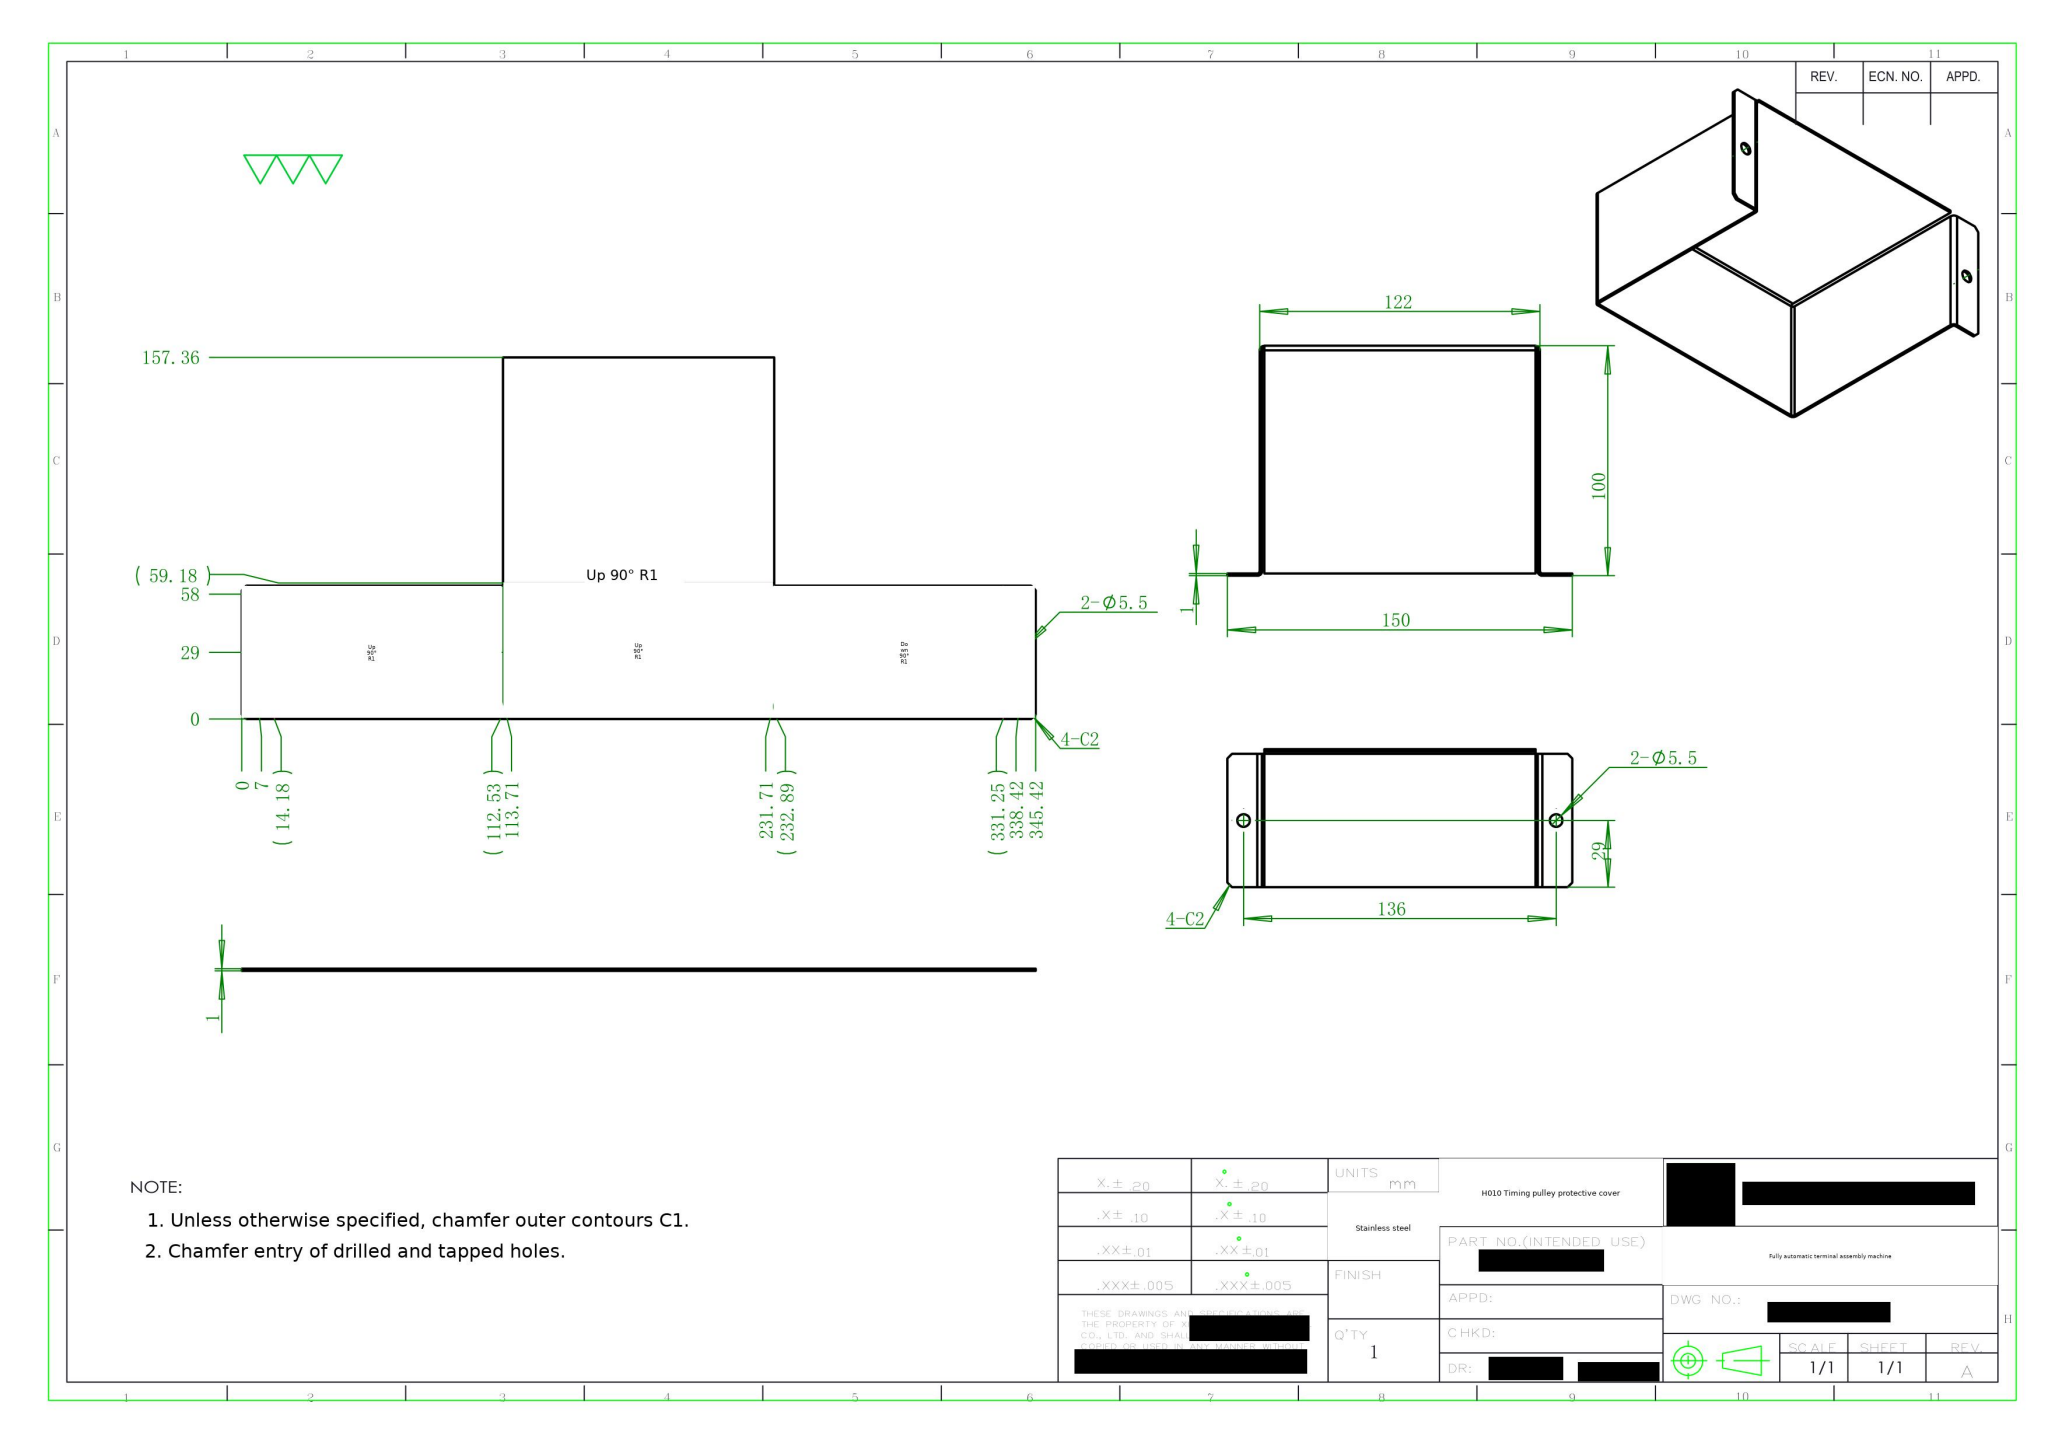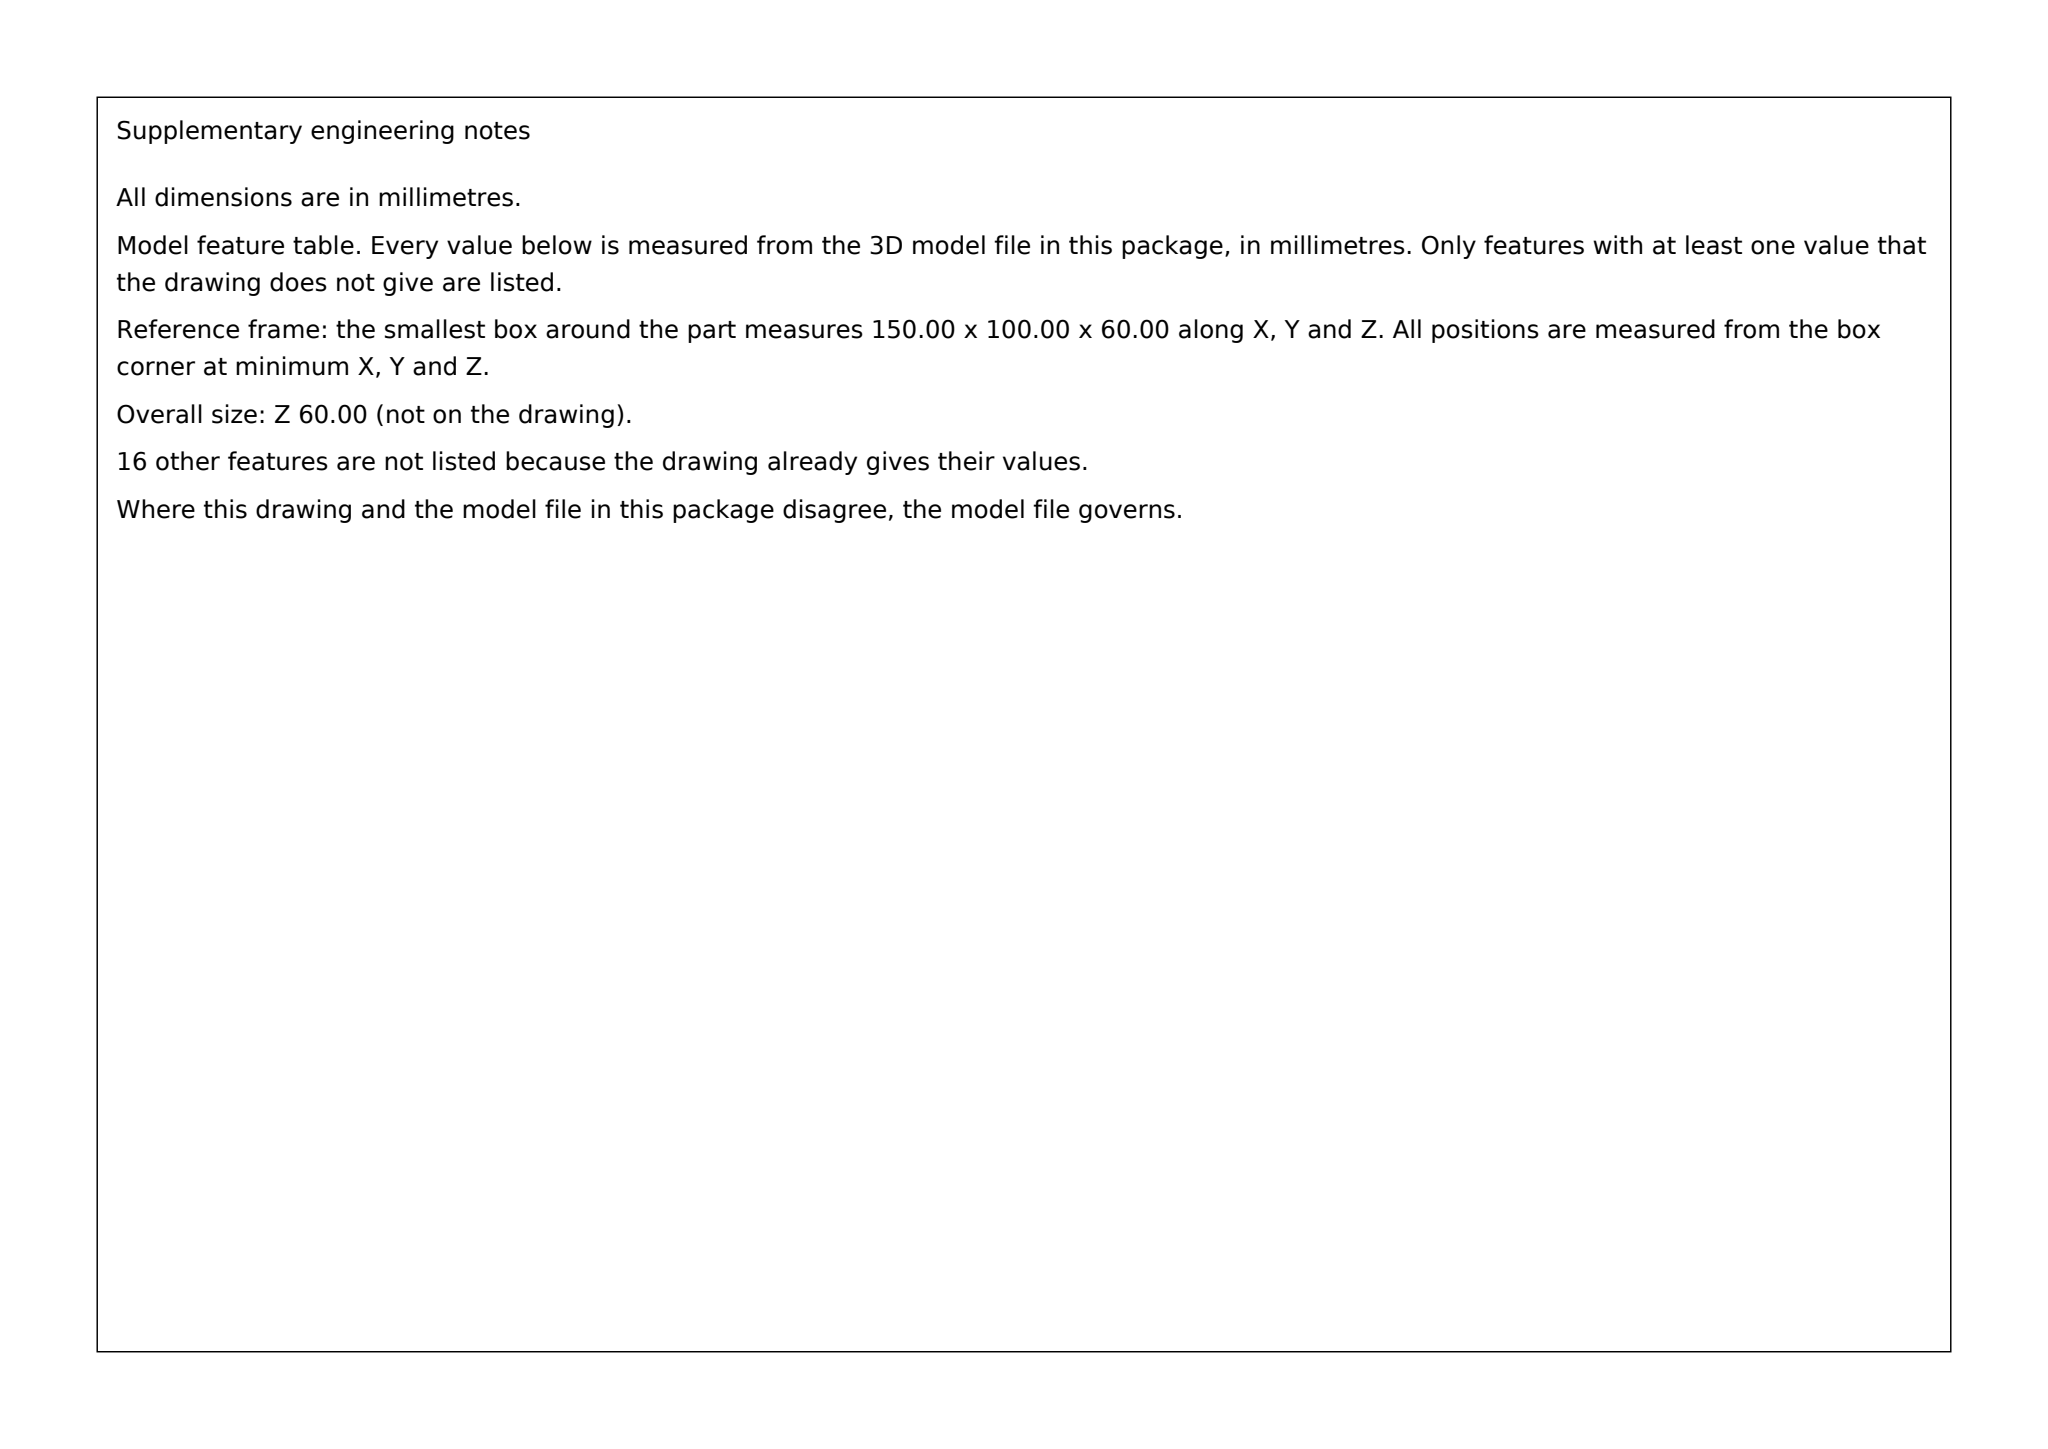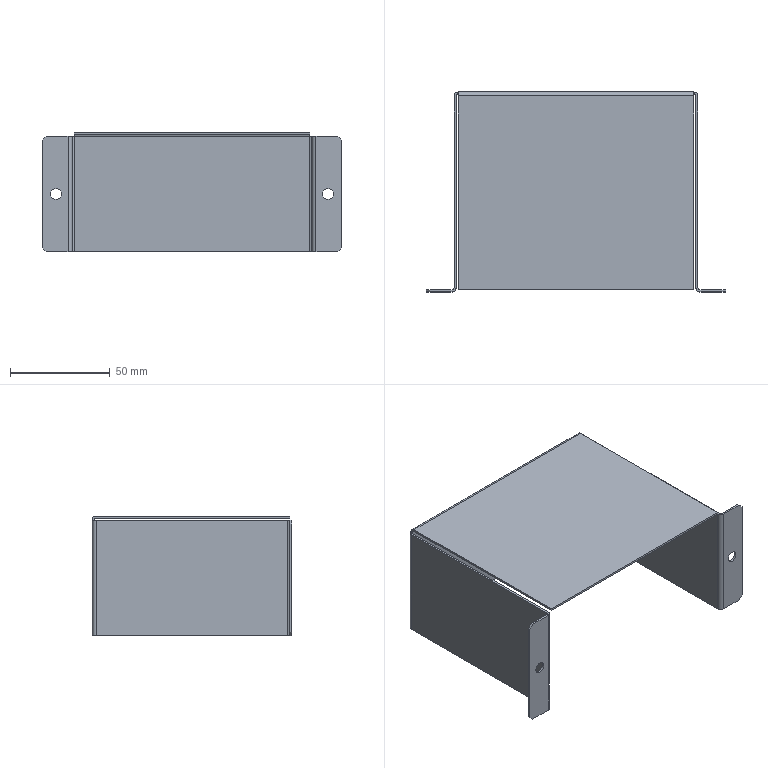Part | SolidWorks | mm | material Stainless steel | 1 solid | 54 faces | box 150 x 100 x 60 mm | volume 31703 mm3 | plane 40 | cylinder 14 | commonest cylinder face diameters 4 x5 2 x5 5.5 x4